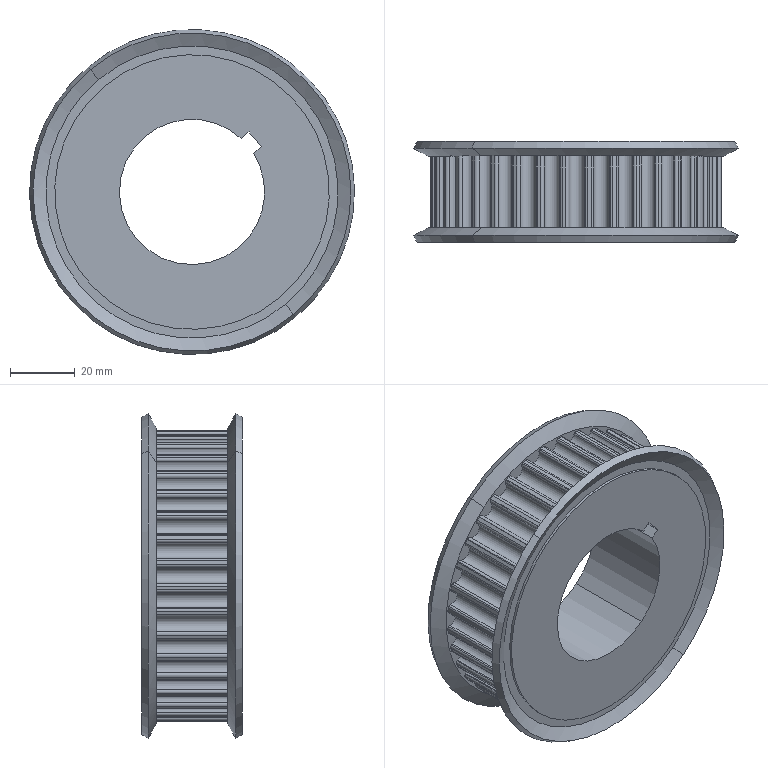Component | SolidWorks | HTS8-36-20A-1 | 1 solid | 207 faces | box 100.69 x 31.2 x 100.69 mm | volume 131838 mm3 | cylinder 186 | cone 12 | plane 9 | commonest cylinder face diameters 1.81 x90 4.8 x53 90.302 x36 85.069 x4 45 x3
build123d program:
from build123d import *

# Parameters (mm, degrees)
TOOTH_EXTRUDE_START = -11.113
TOOTH_EXTRUDE_DEPTH = 22.225
CIRPATTERN1_COUNT   = 36
CUT_EXTRUDE1_DEPTH  = 30


with BuildPart() as part:
    # GearBelt-BaseSketch → HTS 8mm_ 20mm Timing Belt Width_ 91.673 (revolve)
    with BuildSketch(Plane(origin=(0, 0, 0), x_dir=(0, 0, -1), z_dir=(1, 0, 0)), mode=Mode.PRIVATE) as hts_8mm_20mm_timing_belt_width_91_6732_sk:
        Polygon((-14.287, 0), (14.287, 0), (14.287, 42.535), (13.494, 42.535), (13.494, 45.246), (15.599, 49.233), (13.494, 50.345), (11.113, 45.837), (11.113, 45.151), (-11.113, 45.151), (-11.113, 45.837), (-13.494, 50.345), (-15.599, 49.233), (-13.494, 45.246), (-13.494, 42.535), (-14.287, 42.535), align=None)
    revolve(hts_8mm_20mm_timing_belt_width_91_6732_sk.sketch.rotate(Axis((0, 0, 21.431), (0, 0, -1)), 90), axis=Axis((0, 0, 21.431), (0, 0, -1)))

    # Tooth Profile-Sketch → Tooth-Extrude (cut)
    with BuildSketch(Plane.XY.offset(TOOTH_EXTRUDE_START)):
        with BuildLine():
            Line((3.372, 45.025), (0, 47.691))
            Line((0, 47.691), (-3.372, 45.025))
            ThreePointArc((-3.372, 45.025), (-2.689, 44.786), (-2.4, 44.122))
            ThreePointArc((-2.4, 44.122), (0, 41.722), (2.4, 44.122))
            ThreePointArc((2.4, 44.122), (2.689, 44.786), (3.372, 45.025))
        make_face()
    tooth_extrude = extrude(amount=TOOTH_EXTRUDE_DEPTH, mode=Mode.SUBTRACT)

    # CirPattern1: Tooth-Extrude ×36 about axis
    cirpattern1_axis = Axis((0, 0, 0), (0, 0, 1))
    for i in range(1, CIRPATTERN1_COUNT):
        add(tooth_extrude.rotate(cirpattern1_axis, i * 360 / CIRPATTERN1_COUNT), mode=Mode.SUBTRACT)

    # Sketch1 → Cut-Extrude1 (cut)
    with BuildSketch(Plane.XY.offset(14.287)):
        with BuildLine():
            Line((-3, 22.299), (-3, 25.5))
            Line((-3, 25.5), (3, 25.5))
            Line((3, 25.5), (3, 22.299))
            ThreePointArc((3, 22.299), (0, -22.5), (-3, 22.299))
        make_face()
    extrude(amount=-CUT_EXTRUDE1_DEPTH, mode=Mode.SUBTRACT)


solid = part.part

# Placed as in the assembly
solid = solid.moved(Location((-240, 631.966, 90), (-90, 0, -129.731)))